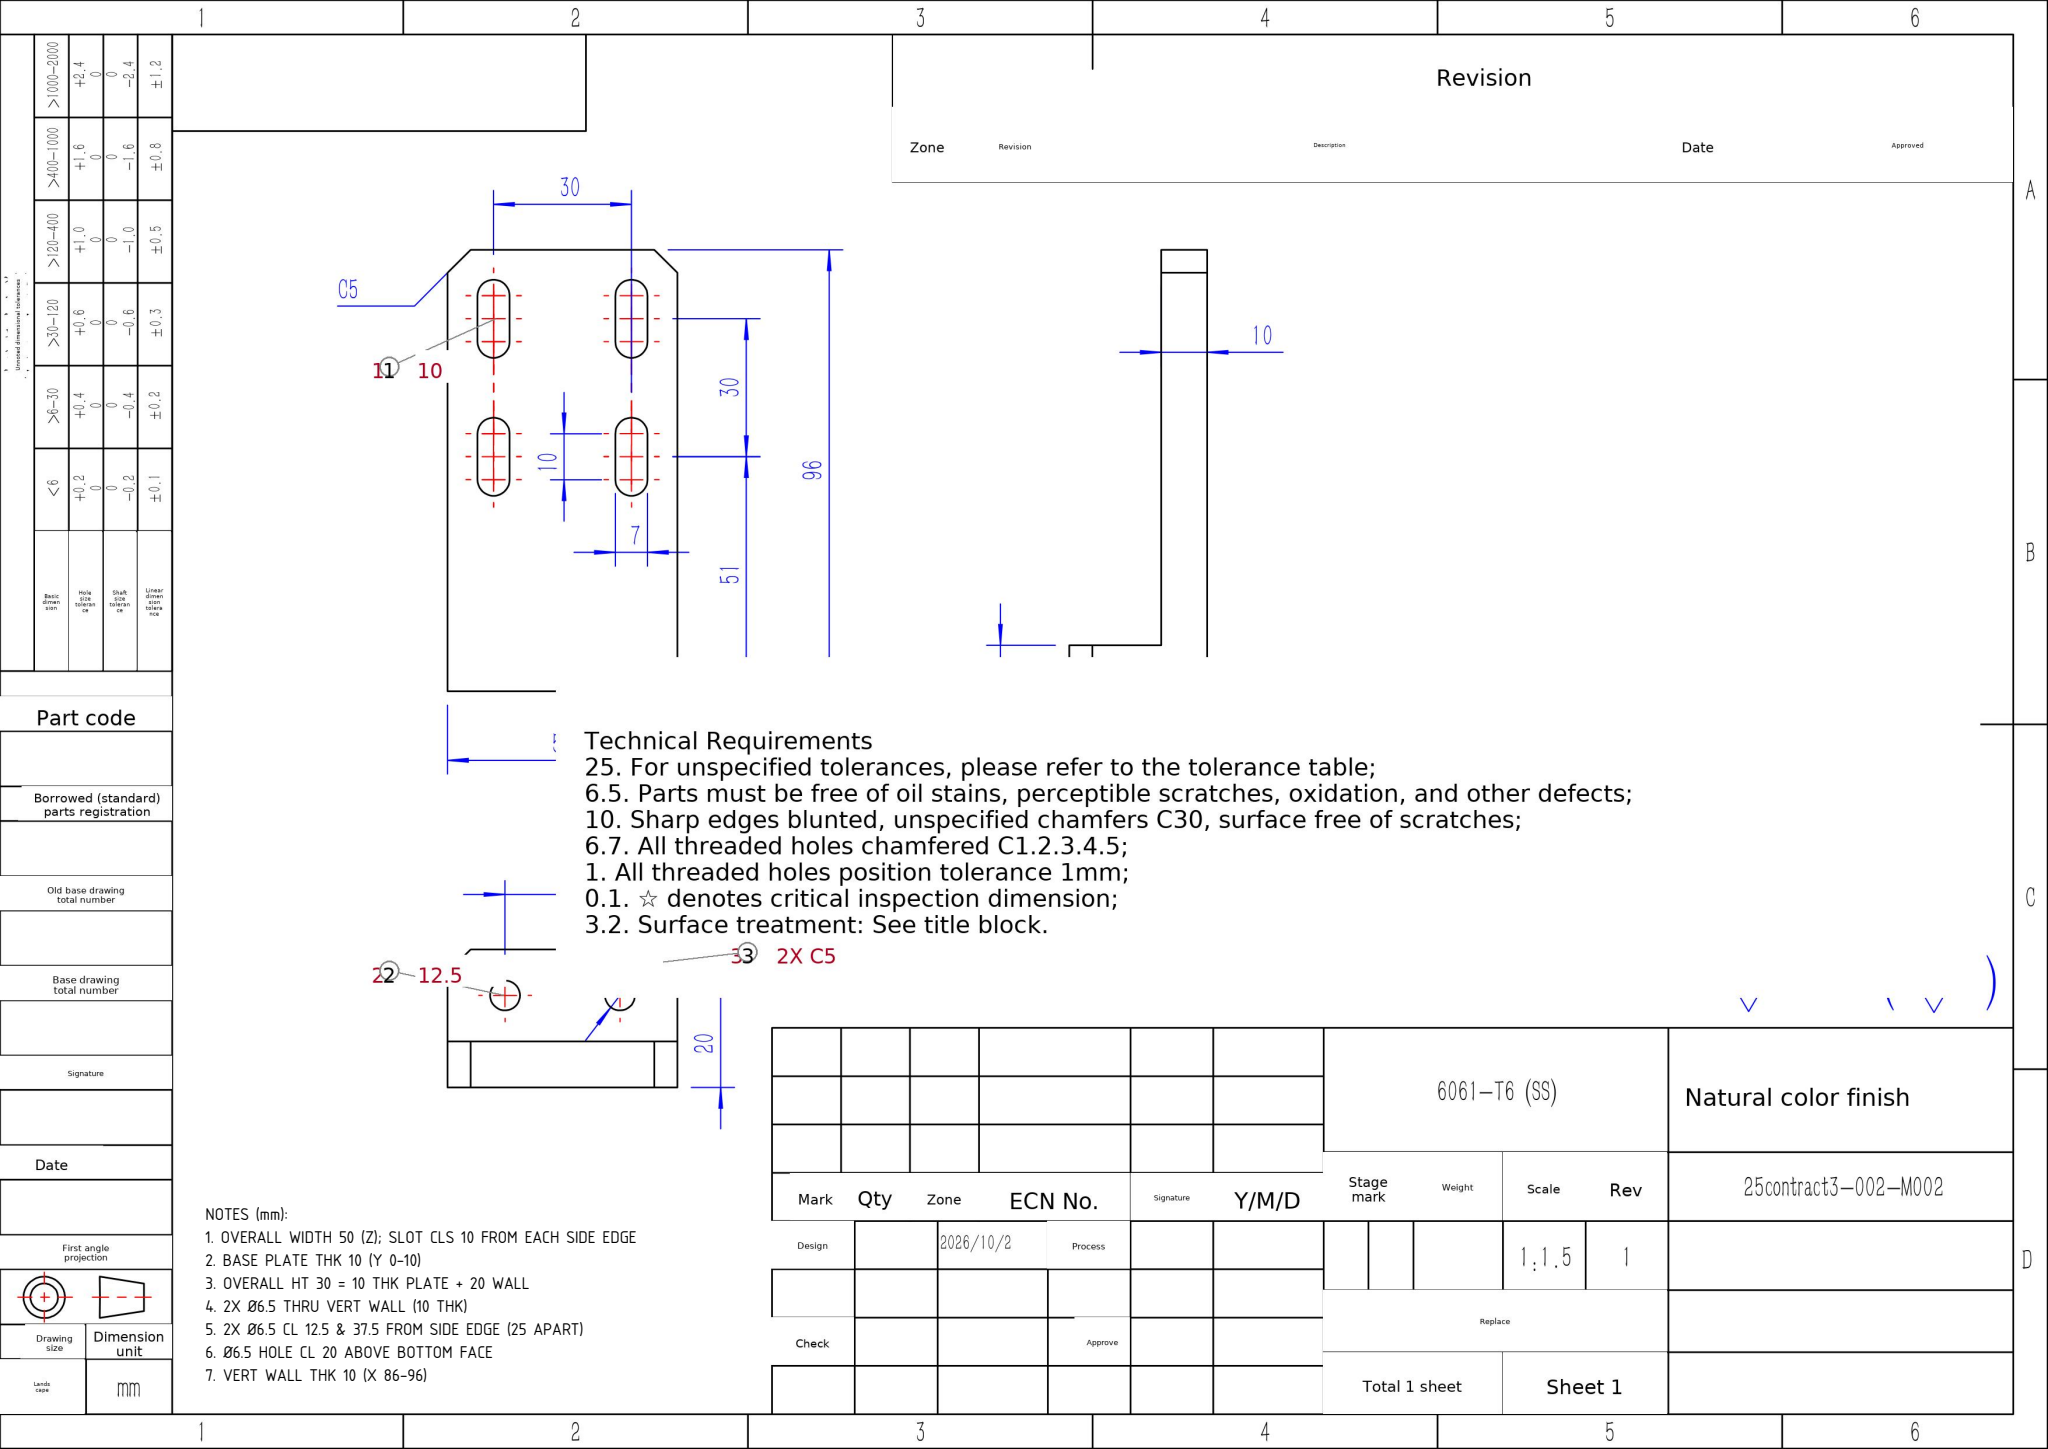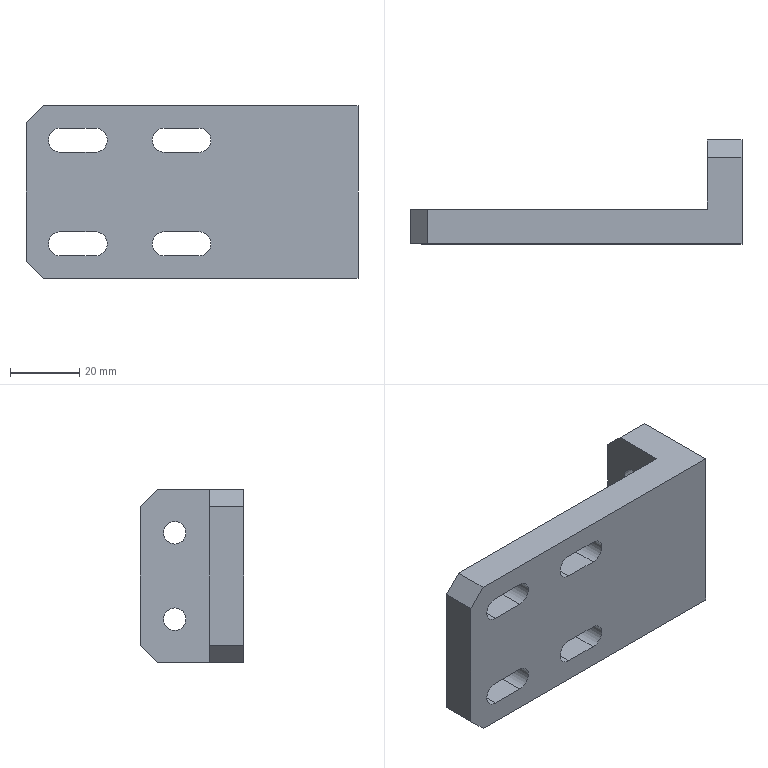Part | SolidWorks | mm | 1 solid | 32 faces | box 96 x 30 x 50 mm | volume 52497 mm3 | plane 20 | cylinder 12 | commonest cylinder face diameters 7 x8 6.5 x4
Drawing notes:
OVERALL WIDTH 50 (Z); SLOT CLS 10 FROM EACH SIDE EDGE | from the solid: bbox Z=50; Ø7 slot axes at z=10 and z=40
BASE PLATE THK 10 (Y 0-10) | from the solid: y planes at 0 and 10; Ø7 slots length 10
OVERALL HT 30 = 10 THK PLATE + 20 WALL | from the solid: y planes 0, 10, 30; bbox Y=30
2X Ø6.5 THRU VERT WALL (10 THK) | from the solid: cyl dia 6.5, axis x, length 10, x wall 86-96
2X Ø6.5 CL 12.5 & 37.5 FROM SIDE EDGE (25 APART) | from the solid: cyl dia 6.5 at z=12.5 and z=37.5
Ø6.5 HOLE CL 20 ABOVE BOTTOM FACE | from the solid: cyl dia 6.5 at y=20; bottom face y=0
VERT WALL THK 10 (X 86-96) | from the solid: x planes at 86.0 and 96.0
STEP:
#1=CARTESIAN_POINT('',(48.,20.,9.25));
#2=VERTEX_POINT('',#1);
#3=CARTESIAN_POINT('',(48.,20.,15.75));
#4=VERTEX_POINT('',#3);
#5=CARTESIAN_POINT('',(48.,20.,12.5));
#6=DIRECTION('',(-1.,0.,-0.));
#7=DIRECTION('',(0.,0.,1.));
#8=AXIS2_PLACEMENT_3D('',#5,#6,#7);
#9=CIRCLE('',#8,3.25);
#10=EDGE_CURVE('',#2,#4,#9,.T.);
#11=ORIENTED_EDGE('',*,*,#10,.F.);
#12=CARTESIAN_POINT('',(38.,20.,9.25));
#13=VERTEX_POINT('',#12);
#14=CARTESIAN_POINT('',(38.,20.,9.25));
#15=DIRECTION('',(-1.,0.,-0.));
#16=VECTOR('',#15,1000.);
#17=LINE('',#14,#16);
#18=EDGE_CURVE('',#2,#13,#17,.T.);
#19=ORIENTED_EDGE('',*,*,#18,.T.);
#20=CARTESIAN_POINT('',(38.,20.,15.75));
#21=VERTEX_POINT('',#20);
#22=CARTESIAN_POINT('',(38.,20.,12.5));
#23=DIRECTION('',(-1.,0.,-0.));
#24=DIRECTION('',(0.,0.,1.));
#25=AXIS2_PLACEMENT_3D('',#22,#23,#24);
#26=CIRCLE('',#25,3.25);
#27=EDGE_CURVE('',#13,#21,#26,.T.);
#28=ORIENTED_EDGE('',*,*,#27,.T.);
#29=CARTESIAN_POINT('',(38.,20.,15.75));
#30=DIRECTION('',(-1.,0.,-0.));
#31=VECTOR('',#30,1000.);
#32=LINE('',#29,#31);
#33=EDGE_CURVE('',#4,#21,#32,.T.);
#34=ORIENTED_EDGE('',*,*,#33,.F.);
#35=EDGE_LOOP('',(#11,#19,#28,#34));
#36=FACE_OUTER_BOUND('',#35,.T.);
#37=CARTESIAN_POINT('',(38.,20.,12.5));
#38=DIRECTION('',(-1.,0.,-0.));
#39=DIRECTION('',(0.,0.,1.));
#40=AXIS2_PLACEMENT_3D('',#37,#38,#39);
#41=CYLINDRICAL_SURFACE('',#40,3.25);
#42=ADVANCED_FACE('',(#36),#41,.F.);
#43=CARTESIAN_POINT('',(48.,20.,-15.75));
#44=VERTEX_POINT('',#43);
#45=CARTESIAN_POINT('',(48.,20.,-9.25));
#46=VERTEX_POINT('',#45);
#47=CARTESIAN_POINT('',(48.,20.,-12.5));
#48=DIRECTION('',(-1.,0.,-0.));
#49=DIRECTION('',(0.,0.,1.));
#50=AXIS2_PLACEMENT_3D('',#47,#48,#49);
#51=CIRCLE('',#50,3.25);
#52=EDGE_CURVE('',#44,#46,#51,.T.);
#53=ORIENTED_EDGE('',*,*,#52,.F.);
#54=CARTESIAN_POINT('',(38.,20.,-15.75));
#55=VERTEX_POINT('',#54);
#56=CARTESIAN_POINT('',(38.,20.,-15.75));
#57=DIRECTION('',(-1.,0.,-0.));
#58=VECTOR('',#57,1000.);
#59=LINE('',#56,#58);
#60=EDGE_CURVE('',#44,#55,#59,.T.);
#61=ORIENTED_EDGE('',*,*,#60,.T.);
#62=CARTESIAN_POINT('',(38.,20.,-9.25));
#63=VERTEX_POINT('',#62);
#64=CARTESIAN_POINT('',(38.,20.,-12.5));
#65=DIRECTION('',(-1.,0.,-0.));
#66=DIRECTION('',(0.,0.,1.));
#67=AXIS2_PLACEMENT_3D('',#64,#65,#66);
#68=CIRCLE('',#67,3.25);
#69=EDGE_CURVE('',#55,#63,#68,.T.);
#70=ORIENTED_EDGE('',*,*,#69,.T.);
#71=CARTESIAN_POINT('',(38.,20.,-9.25));
#72=DIRECTION('',(-1.,0.,-0.));
#73=VECTOR('',#72,1000.);
#74=LINE('',#71,#73);
#75=EDGE_CURVE('',#46,#63,#74,.T.);
#76=ORIENTED_EDGE('',*,*,#75,.F.);
#77=EDGE_LOOP('',(#53,#61,#70,#76));
#78=FACE_OUTER_BOUND('',#77,.T.);
#79=CARTESIAN_POINT('',(38.,20.,-12.5));
#80=DIRECTION('',(-1.,0.,-0.));
#81=DIRECTION('',(0.,0.,1.));
#82=AXIS2_PLACEMENT_3D('',#79,#80,#81);
#83=CYLINDRICAL_SURFACE('',#82,3.25);
#84=ADVANCED_FACE('',(#78),#83,.F.);
#85=CARTESIAN_POINT('',(48.,20.,12.5));
#86=DIRECTION('',(-1.,0.,-0.));
#87=DIRECTION('',(0.,0.,1.));
#88=AXIS2_PLACEMENT_3D('',#85,#86,#87);
#89=CIRCLE('',#88,3.25);
#90=EDGE_CURVE('',#4,#2,#89,.T.);
#91=ORIENTED_EDGE('',*,*,#90,.T.);
#92=ORIENTED_EDGE('',*,*,#10,.T.);
#93=EDGE_LOOP('',(#91,#92));
#94=FACE_BOUND('',#93,.T.);
#95=CARTESIAN_POINT('',(48.,20.,-12.5));
#96=DIRECTION('',(-1.,0.,-0.));
#97=DIRECTION('',(0.,0.,1.));
#98=AXIS2_PLACEMENT_3D('',#95,#96,#97);
#99=CIRCLE('',#98,3.25);
#100=EDGE_CURVE('',#46,#44,#99,.T.);
#101=ORIENTED_EDGE('',*,*,#100,.T.);
#102=ORIENTED_EDGE('',*,*,#52,.T.);
#103=EDGE_LOOP('',(#101,#102));
#104=FACE_BOUND('',#103,.T.);
#105=CARTESIAN_POINT('',(48.,30.,-20.));
#106=VERTEX_POINT('',#105);
#107=CARTESIAN_POINT('',(48.,30.,20.));
#108=VERTEX_POINT('',#107);
#109=CARTESIAN_POINT('',(48.,30.,-25.));
#110=DIRECTION('',(0.,0.,1.));
#111=VECTOR('',#110,1000.);
#112=LINE('',#109,#111);
#113=EDGE_CURVE('',#106,#108,#112,.T.);
#114=ORIENTED_EDGE('',*,*,#113,.T.);
#115=CARTESIAN_POINT('',(48.,25.,25.));
#116=VERTEX_POINT('',#115);
#117=CARTESIAN_POINT('',(48.,25.,25.));
#118=DIRECTION('',(0.,-0.7071,0.7071));
#119=VECTOR('',#118,1000.);
#120=LINE('',#117,#119);
#121=EDGE_CURVE('',#108,#116,#120,.T.);
#122=ORIENTED_EDGE('',*,*,#121,.T.);
#123=CARTESIAN_POINT('',(48.,0.,25.));
#124=VERTEX_POINT('',#123);
#125=CARTESIAN_POINT('',(48.,10.,25.));
#126=DIRECTION('',(0.,-1.,0.));
#127=VECTOR('',#126,1000.);
#128=LINE('',#125,#127);
#129=EDGE_CURVE('',#116,#124,#128,.T.);
#130=ORIENTED_EDGE('',*,*,#129,.T.);
#131=CARTESIAN_POINT('',(48.,0.,-25.));
#132=VERTEX_POINT('',#131);
#133=CARTESIAN_POINT('',(48.,0.,25.));
#134=DIRECTION('',(0.,0.,-1.));
#135=VECTOR('',#134,1000.);
#136=LINE('',#133,#135);
#137=EDGE_CURVE('',#124,#132,#136,.T.);
#138=ORIENTED_EDGE('',*,*,#137,.T.);
#139=CARTESIAN_POINT('',(48.,25.,-25.));
#140=VERTEX_POINT('',#139);
#141=CARTESIAN_POINT('',(48.,10.,-25.));
#142=DIRECTION('',(0.,-1.,0.));
#143=VECTOR('',#142,1000.);
#144=LINE('',#141,#143);
#145=EDGE_CURVE('',#140,#132,#144,.T.);
#146=ORIENTED_EDGE('',*,*,#145,.F.);
#147=CARTESIAN_POINT('',(48.,25.,-25.));
#148=DIRECTION('',(0.,0.7071,0.7071));
#149=VECTOR('',#148,1000.);
#150=LINE('',#147,#149);
#151=EDGE_CURVE('',#140,#106,#150,.T.);
#152=ORIENTED_EDGE('',*,*,#151,.T.);
#153=EDGE_LOOP('',(#114,#122,#130,#138,#146,#152));
#154=FACE_OUTER_BOUND('',#153,.T.);
#155=CARTESIAN_POINT('',(48.,10.,25.));
#156=DIRECTION('',(-1.,0.,0.));
#157=DIRECTION('',(0.,0.,1.));
#158=AXIS2_PLACEMENT_3D('',#155,#156,#157);
#159=PLANE('',#158);
#160=ADVANCED_FACE('',(#94,#104,#154),#159,.F.);
#161=CARTESIAN_POINT('',(38.,25.,-25.));
#162=VERTEX_POINT('',#161);
#163=CARTESIAN_POINT('',(38.,10.,-25.));
#164=VERTEX_POINT('',#163);
#165=CARTESIAN_POINT('',(38.,30.,-25.));
#166=DIRECTION('',(0.,-1.,0.));
#167=VECTOR('',#166,1000.);
#168=LINE('',#165,#167);
#169=EDGE_CURVE('',#162,#164,#168,.T.);
#170=ORIENTED_EDGE('',*,*,#169,.F.);
#171=CARTESIAN_POINT('',(-48.,25.,-25.));
#172=DIRECTION('',(1.,0.,0.));
#173=VECTOR('',#172,1000.);
#174=LINE('',#171,#173);
#175=EDGE_CURVE('',#162,#140,#174,.T.);
#176=ORIENTED_EDGE('',*,*,#175,.T.);
#177=ORIENTED_EDGE('',*,*,#145,.T.);
#178=CARTESIAN_POINT('',(-43.,0.,-25.));
#179=VERTEX_POINT('',#178);
#180=CARTESIAN_POINT('',(-48.,0.,-25.));
#181=DIRECTION('',(-1.,0.,0.));
#182=VECTOR('',#181,1000.);
#183=LINE('',#180,#182);
#184=EDGE_CURVE('',#132,#179,#183,.T.);
#185=ORIENTED_EDGE('',*,*,#184,.T.);
#186=CARTESIAN_POINT('',(-43.,10.,-25.));
#187=VERTEX_POINT('',#186);
#188=CARTESIAN_POINT('',(-43.,10.,-25.));
#189=DIRECTION('',(0.,1.,0.));
#190=VECTOR('',#189,1000.);
#191=LINE('',#188,#190);
#192=EDGE_CURVE('',#179,#187,#191,.T.);
#193=ORIENTED_EDGE('',*,*,#192,.T.);
#194=CARTESIAN_POINT('',(-48.,10.,-25.));
#195=DIRECTION('',(-1.,0.,0.));
#196=VECTOR('',#195,1000.);
#197=LINE('',#194,#196);
#198=EDGE_CURVE('',#164,#187,#197,.T.);
#199=ORIENTED_EDGE('',*,*,#198,.F.);
#200=EDGE_LOOP('',(#170,#176,#177,#185,#193,#199));
#201=FACE_OUTER_BOUND('',#200,.T.);
#202=CARTESIAN_POINT('',(-48.,10.,-25.));
#203=DIRECTION('',(0.,0.,1.));
#204=DIRECTION('',(1.,0.,0.));
#205=AXIS2_PLACEMENT_3D('',#202,#203,#204);
#206=PLANE('',#205);
#207=ADVANCED_FACE('',(#201),#206,.F.);
#208=CARTESIAN_POINT('',(-48.,10.,-20.));
#209=VERTEX_POINT('',#208);
#210=CARTESIAN_POINT('',(-48.,10.,20.));
#211=VERTEX_POINT('',#210);
#212=CARTESIAN_POINT('',(-48.,10.,25.));
#213=DIRECTION('',(0.,0.,1.));
#214=VECTOR('',#213,1000.);
#215=LINE('',#212,#214);
#216=EDGE_CURVE('',#209,#211,#215,.T.);
#217=ORIENTED_EDGE('',*,*,#216,.F.);
#218=CARTESIAN_POINT('',(-48.,0.,-20.));
#219=VERTEX_POINT('',#218);
#220=CARTESIAN_POINT('',(-48.,10.,-20.));
#221=DIRECTION('',(0.,-1.,0.));
#222=VECTOR('',#221,1000.);
#223=LINE('',#220,#222);
#224=EDGE_CURVE('',#209,#219,#223,.T.);
#225=ORIENTED_EDGE('',*,*,#224,.T.);
#226=CARTESIAN_POINT('',(-48.,0.,20.));
#227=VERTEX_POINT('',#226);
#228=CARTESIAN_POINT('',(-48.,0.,25.));
#229=DIRECTION('',(0.,0.,1.));
#230=VECTOR('',#229,1000.);
#231=LINE('',#228,#230);
#232=EDGE_CURVE('',#219,#227,#231,.T.);
#233=ORIENTED_EDGE('',*,*,#232,.T.);
#234=CARTESIAN_POINT('',(-48.,10.,20.));
#235=DIRECTION('',(0.,1.,0.));
#236=VECTOR('',#235,1000.);
#237=LINE('',#234,#236);
#238=EDGE_CURVE('',#227,#211,#237,.T.);
#239=ORIENTED_EDGE('',*,*,#238,.T.);
#240=EDGE_LOOP('',(#217,#225,#233,#239));
#241=FACE_OUTER_BOUND('',#240,.T.);
#242=CARTESIAN_POINT('',(-48.,10.,25.));
#243=DIRECTION('',(1.,0.,0.));
#244=DIRECTION('',(0.,0.,-1.));
#245=AXIS2_PLACEMENT_3D('',#242,#243,#244);
#246=PLANE('',#245);
#247=ADVANCED_FACE('',(#241),#246,.F.);
#248=ORIENTED_EDGE('',*,*,#129,.F.);
#249=CARTESIAN_POINT('',(38.,25.,25.));
#250=VERTEX_POINT('',#249);
#251=CARTESIAN_POINT('',(-48.,25.,25.));
#252=DIRECTION('',(-1.,0.,0.));
#253=VECTOR('',#252,1000.);
#254=LINE('',#251,#253);
#255=EDGE_CURVE('',#116,#250,#254,.T.);
#256=ORIENTED_EDGE('',*,*,#255,.T.);
#257=CARTESIAN_POINT('',(38.,10.,25.));
#258=VERTEX_POINT('',#257);
#259=CARTESIAN_POINT('',(38.,30.,25.));
#260=DIRECTION('',(0.,-1.,0.));
#261=VECTOR('',#260,1000.);
#262=LINE('',#259,#261);
#263=EDGE_CURVE('',#250,#258,#262,.T.);
#264=ORIENTED_EDGE('',*,*,#263,.T.);
#265=CARTESIAN_POINT('',(-43.,10.,25.));
#266=VERTEX_POINT('',#265);
#267=CARTESIAN_POINT('',(-48.,10.,25.));
#268=DIRECTION('',(1.,0.,0.));
#269=VECTOR('',#268,1000.);
#270=LINE('',#267,#269);
#271=EDGE_CURVE('',#266,#258,#270,.T.);
#272=ORIENTED_EDGE('',*,*,#271,.F.);
#273=CARTESIAN_POINT('',(-43.,0.,25.));
#274=VERTEX_POINT('',#273);
#275=CARTESIAN_POINT('',(-43.,10.,25.));
#276=DIRECTION('',(0.,-1.,0.));
#277=VECTOR('',#276,1000.);
#278=LINE('',#275,#277);
#279=EDGE_CURVE('',#266,#274,#278,.T.);
#280=ORIENTED_EDGE('',*,*,#279,.T.);
#281=CARTESIAN_POINT('',(-48.,0.,25.));
#282=DIRECTION('',(1.,0.,0.));
#283=VECTOR('',#282,1000.);
#284=LINE('',#281,#283);
#285=EDGE_CURVE('',#274,#124,#284,.T.);
#286=ORIENTED_EDGE('',*,*,#285,.T.);
#287=EDGE_LOOP('',(#248,#256,#264,#272,#280,#286));
#288=FACE_OUTER_BOUND('',#287,.T.);
#289=CARTESIAN_POINT('',(-48.,10.,25.));
#290=DIRECTION('',(0.,0.,-1.));
#291=DIRECTION('',(-1.,0.,0.));
#292=AXIS2_PLACEMENT_3D('',#289,#290,#291);
#293=PLANE('',#292);
#294=ADVANCED_FACE('',(#288),#293,.F.);
#295=CARTESIAN_POINT('',(-8.,10.,18.5));
#296=VERTEX_POINT('',#295);
#297=CARTESIAN_POINT('',(2.,10.,18.5));
#298=VERTEX_POINT('',#297);
#299=CARTESIAN_POINT('',(-8.,10.,18.5));
#300=DIRECTION('',(1.,0.,0.));
#301=VECTOR('',#300,1000.);
#302=LINE('',#299,#301);
#303=EDGE_CURVE('',#296,#298,#302,.T.);
#304=ORIENTED_EDGE('',*,*,#303,.F.);
#305=CARTESIAN_POINT('',(-8.,10.,11.5));
#306=VERTEX_POINT('',#305);
#307=CARTESIAN_POINT('',(-8.,10.,15.));
#308=DIRECTION('',(0.,1.,0.));
#309=DIRECTION('',(0.,0.,1.));
#310=AXIS2_PLACEMENT_3D('',#307,#308,#309);
#311=CIRCLE('',#310,3.5);
#312=EDGE_CURVE('',#306,#296,#311,.T.);
#313=ORIENTED_EDGE('',*,*,#312,.F.);
#314=CARTESIAN_POINT('',(2.,10.,11.5));
#315=VERTEX_POINT('',#314);
#316=CARTESIAN_POINT('',(-8.,10.,11.5));
#317=DIRECTION('',(-1.,0.,0.));
#318=VECTOR('',#317,1000.);
#319=LINE('',#316,#318);
#320=EDGE_CURVE('',#315,#306,#319,.T.);
#321=ORIENTED_EDGE('',*,*,#320,.F.);
#322=CARTESIAN_POINT('',(2.,10.,15.));
#323=DIRECTION('',(0.,1.,0.));
#324=DIRECTION('',(0.,0.,1.));
#325=AXIS2_PLACEMENT_3D('',#322,#323,#324);
#326=CIRCLE('',#325,3.5);
#327=EDGE_CURVE('',#298,#315,#326,.T.);
#328=ORIENTED_EDGE('',*,*,#327,.F.);
#329=EDGE_LOOP('',(#304,#313,#321,#328));
#330=FACE_BOUND('',#329,.T.);
#331=CARTESIAN_POINT('',(-8.,10.,-11.5));
#332=VERTEX_POINT('',#331);
#333=CARTESIAN_POINT('',(2.,10.,-11.5));
#334=VERTEX_POINT('',#333);
#335=CARTESIAN_POINT('',(-8.,10.,-11.5));
#336=DIRECTION('',(1.,0.,0.));
#337=VECTOR('',#336,1000.);
#338=LINE('',#335,#337);
#339=EDGE_CURVE('',#332,#334,#338,.T.);
#340=ORIENTED_EDGE('',*,*,#339,.F.);
#341=CARTESIAN_POINT('',(-8.,10.,-18.5));
#342=VERTEX_POINT('',#341);
#343=CARTESIAN_POINT('',(-8.,10.,-15.));
#344=DIRECTION('',(0.,1.,0.));
#345=DIRECTION('',(0.,0.,-1.));
#346=AXIS2_PLACEMENT_3D('',#343,#344,#345);
#347=CIRCLE('',#346,3.5);
#348=EDGE_CURVE('',#342,#332,#347,.T.);
#349=ORIENTED_EDGE('',*,*,#348,.F.);
#350=CARTESIAN_POINT('',(2.,10.,-18.5));
#351=VERTEX_POINT('',#350);
#352=CARTESIAN_POINT('',(-8.,10.,-18.5));
#353=DIRECTION('',(-1.,0.,0.));
#354=VECTOR('',#353,1000.);
#355=LINE('',#352,#354);
#356=EDGE_CURVE('',#351,#342,#355,.T.);
#357=ORIENTED_EDGE('',*,*,#356,.F.);
#358=CARTESIAN_POINT('',(2.,10.,-15.));
#359=DIRECTION('',(0.,1.,0.));
#360=DIRECTION('',(0.,0.,-1.));
#361=AXIS2_PLACEMENT_3D('',#358,#359,#360);
#362=CIRCLE('',#361,3.5);
#363=EDGE_CURVE('',#334,#351,#362,.T.);
#364=ORIENTED_EDGE('',*,*,#363,.F.);
#365=EDGE_LOOP('',(#340,#349,#357,#364));
#366=FACE_BOUND('',#365,.T.);
#367=CARTESIAN_POINT('',(-38.,10.,18.5));
#368=VERTEX_POINT('',#367);
#369=CARTESIAN_POINT('',(-28.,10.,18.5));
#370=VERTEX_POINT('',#369);
#371=CARTESIAN_POINT('',(-38.,10.,18.5));
#372=DIRECTION('',(1.,0.,0.));
#373=VECTOR('',#372,1000.);
#374=LINE('',#371,#373);
#375=EDGE_CURVE('',#368,#370,#374,.T.);
#376=ORIENTED_EDGE('',*,*,#375,.F.);
#377=CARTESIAN_POINT('',(-38.,10.,11.5));
#378=VERTEX_POINT('',#377);
#379=CARTESIAN_POINT('',(-38.,10.,15.));
#380=DIRECTION('',(0.,1.,0.));
#381=DIRECTION('',(0.,0.,1.));
#382=AXIS2_PLACEMENT_3D('',#379,#380,#381);
#383=CIRCLE('',#382,3.5);
#384=EDGE_CURVE('',#378,#368,#383,.T.);
#385=ORIENTED_EDGE('',*,*,#384,.F.);
#386=CARTESIAN_POINT('',(-28.,10.,11.5));
#387=VERTEX_POINT('',#386);
#388=CARTESIAN_POINT('',(-38.,10.,11.5));
#389=DIRECTION('',(-1.,0.,0.));
#390=VECTOR('',#389,1000.);
#391=LINE('',#388,#390);
#392=EDGE_CURVE('',#387,#378,#391,.T.);
#393=ORIENTED_EDGE('',*,*,#392,.F.);
#394=CARTESIAN_POINT('',(-28.,10.,15.));
#395=DIRECTION('',(0.,1.,0.));
#396=DIRECTION('',(0.,0.,1.));
#397=AXIS2_PLACEMENT_3D('',#394,#395,#396);
#398=CIRCLE('',#397,3.5);
#399=EDGE_CURVE('',#370,#387,#398,.T.);
#400=ORIENTED_EDGE('',*,*,#399,.F.);
#401=EDGE_LOOP('',(#376,#385,#393,#400));
#402=FACE_BOUND('',#401,.T.);
#403=CARTESIAN_POINT('',(-38.,10.,-11.5));
#404=VERTEX_POINT('',#403);
#405=CARTESIAN_POINT('',(-28.,10.,-11.5));
#406=VERTEX_POINT('',#405);
#407=CARTESIAN_POINT('',(-38.,10.,-11.5));
#408=DIRECTION('',(1.,0.,0.));
#409=VECTOR('',#408,1000.);
#410=LINE('',#407,#409);
#411=EDGE_CURVE('',#404,#406,#410,.T.);
#412=ORIENTED_EDGE('',*,*,#411,.F.);
#413=CARTESIAN_POINT('',(-38.,10.,-18.5));
#414=VERTEX_POINT('',#413);
#415=CARTESIAN_POINT('',(-38.,10.,-15.));
#416=DIRECTION('',(0.,1.,0.));
#417=DIRECTION('',(0.,0.,-1.));
#418=AXIS2_PLACEMENT_3D('',#415,#416,#417);
#419=CIRCLE('',#418,3.5);
#420=EDGE_CURVE('',#414,#404,#419,.T.);
#421=ORIENTED_EDGE('',*,*,#420,.F.);
#422=CARTESIAN_POINT('',(-28.,10.,-18.5));
#423=VERTEX_POINT('',#422);
#424=CARTESIAN_POINT('',(-38.,10.,-18.5));
#425=DIRECTION('',(-1.,0.,0.));
#426=VECTOR('',#425,1000.);
#427=LINE('',#424,#426);
#428=EDGE_CURVE('',#423,#414,#427,.T.);
#429=ORIENTED_EDGE('',*,*,#428,.F.);
#430=CARTESIAN_POINT('',(-28.,10.,-15.));
#431=DIRECTION('',(0.,1.,0.));
#432=DIRECTION('',(0.,0.,-1.));
#433=AXIS2_PLACEMENT_3D('',#430,#431,#432);
#434=CIRCLE('',#433,3.5);
#435=EDGE_CURVE('',#406,#423,#434,.T.);
#436=ORIENTED_EDGE('',*,*,#435,.F.);
#437=EDGE_LOOP('',(#412,#421,#429,#436));
#438=FACE_BOUND('',#437,.T.);
#439=ORIENTED_EDGE('',*,*,#198,.T.);
#440=CARTESIAN_POINT('',(-48.,10.,-20.));
#441=DIRECTION('',(-0.7071,0.,0.7071));
#442=VECTOR('',#441,1000.);
#443=LINE('',#440,#442);
#444=EDGE_CURVE('',#187,#209,#443,.T.);
#445=ORIENTED_EDGE('',*,*,#444,.T.);
#446=ORIENTED_EDGE('',*,*,#216,.T.);
#447=CARTESIAN_POINT('',(-43.,10.,25.));
#448=DIRECTION('',(0.7071,0.,0.7071));
#449=VECTOR('',#448,1000.);
#450=LINE('',#447,#449);
#451=EDGE_CURVE('',#211,#266,#450,.T.);
#452=ORIENTED_EDGE('',*,*,#451,.T.);
#453=ORIENTED_EDGE('',*,*,#271,.T.);
#454=CARTESIAN_POINT('',(38.,10.,0.));
#455=DIRECTION('',(0.,0.,-1.));
#456=VECTOR('',#455,1000.);
#457=LINE('',#454,#456);
#458=EDGE_CURVE('',#258,#164,#457,.T.);
#459=ORIENTED_EDGE('',*,*,#458,.T.);
#460=EDGE_LOOP('',(#439,#445,#446,#452,#453,#459));
#461=FACE_OUTER_BOUND('',#460,.T.);
#462=CARTESIAN_POINT('',(0.,10.,0.));
#463=DIRECTION('',(0.,-1.,0.));
#464=DIRECTION('',(0.,0.,-1.));
#465=AXIS2_PLACEMENT_3D('',#462,#463,#464);
#466=PLANE('',#465);
#467=ADVANCED_FACE('',(#330,#366,#402,#438,#461),#466,.F.);
#468=CARTESIAN_POINT('',(-8.,0.,11.5));
#469=VERTEX_POINT('',#468);
#470=CARTESIAN_POINT('',(-8.,0.,18.5));
#471=VERTEX_POINT('',#470);
#472=CARTESIAN_POINT('',(-8.,0.,15.));
#473=DIRECTION('',(0.,1.,0.));
#474=DIRECTION('',(0.,0.,1.));
#475=AXIS2_PLACEMENT_3D('',#472,#473,#474);
#476=CIRCLE('',#475,3.5);
#477=EDGE_CURVE('',#469,#471,#476,.T.);
#478=ORIENTED_EDGE('',*,*,#477,.T.);
#479=CARTESIAN_POINT('',(2.,0.,18.5));
#480=VERTEX_POINT('',#479);
#481=CARTESIAN_POINT('',(-8.,0.,18.5));
#482=DIRECTION('',(1.,0.,0.));
#483=VECTOR('',#482,1000.);
#484=LINE('',#481,#483);
#485=EDGE_CURVE('',#471,#480,#484,.T.);
#486=ORIENTED_EDGE('',*,*,#485,.T.);
#487=CARTESIAN_POINT('',(2.,0.,11.5));
#488=VERTEX_POINT('',#487);
#489=CARTESIAN_POINT('',(2.,0.,15.));
#490=DIRECTION('',(0.,1.,0.));
#491=DIRECTION('',(0.,0.,1.));
#492=AXIS2_PLACEMENT_3D('',#489,#490,#491);
#493=CIRCLE('',#492,3.5);
#494=EDGE_CURVE('',#480,#488,#493,.T.);
#495=ORIENTED_EDGE('',*,*,#494,.T.);
#496=CARTESIAN_POINT('',(-8.,0.,11.5));
#497=DIRECTION('',(-1.,0.,0.));
#498=VECTOR('',#497,1000.);
#499=LINE('',#496,#498);
#500=EDGE_CURVE('',#488,#469,#499,.T.);
#501=ORIENTED_EDGE('',*,*,#500,.T.);
#502=EDGE_LOOP('',(#478,#486,#495,#501));
#503=FACE_BOUND('',#502,.T.);
#504=CARTESIAN_POINT('',(-8.,0.,-18.5));
#505=VERTEX_POINT('',#504);
#506=CARTESIAN_POINT('',(-8.,0.,-11.5));
#507=VERTEX_POINT('',#506);
#508=CARTESIAN_POINT('',(-8.,0.,-15.));
#509=DIRECTION('',(0.,1.,0.));
#510=DIRECTION('',(0.,0.,-1.));
#511=AXIS2_PLACEMENT_3D('',#508,#509,#510);
#512=CIRCLE('',#511,3.5);
#513=EDGE_CURVE('',#505,#507,#512,.T.);
#514=ORIENTED_EDGE('',*,*,#513,.T.);
#515=CARTESIAN_POINT('',(2.,0.,-11.5));
#516=VERTEX_POINT('',#515);
#517=CARTESIAN_POINT('',(-8.,0.,-11.5));
#518=DIRECTION('',(1.,0.,0.));
#519=VECTOR('',#518,1000.);
#520=LINE('',#517,#519);
#521=EDGE_CURVE('',#507,#516,#520,.T.);
#522=ORIENTED_EDGE('',*,*,#521,.T.);
#523=CARTESIAN_POINT('',(2.,0.,-18.5));
#524=VERTEX_POINT('',#523);
#525=CARTESIAN_POINT('',(2.,0.,-15.));
#526=DIRECTION('',(0.,1.,0.));
#527=DIRECTION('',(0.,0.,-1.));
#528=AXIS2_PLACEMENT_3D('',#525,#526,#527);
#529=CIRCLE('',#528,3.5);
#530=EDGE_CURVE('',#516,#524,#529,.T.);
#531=ORIENTED_EDGE('',*,*,#530,.T.);
#532=CARTESIAN_POINT('',(-8.,0.,-18.5));
#533=DIRECTION('',(-1.,0.,0.));
#534=VECTOR('',#533,1000.);
#535=LINE('',#532,#534);
#536=EDGE_CURVE('',#524,#505,#535,.T.);
#537=ORIENTED_EDGE('',*,*,#536,.T.);
#538=EDGE_LOOP('',(#514,#522,#531,#537));
#539=FACE_BOUND('',#538,.T.);
#540=CARTESIAN_POINT('',(-38.,0.,11.5));
#541=VERTEX_POINT('',#540);
#542=CARTESIAN_POINT('',(-38.,0.,18.5));
#543=VERTEX_POINT('',#542);
#544=CARTESIAN_POINT('',(-38.,0.,15.));
#545=DIRECTION('',(0.,1.,0.));
#546=DIRECTION('',(0.,0.,1.));
#547=AXIS2_PLACEMENT_3D('',#544,#545,#546);
#548=CIRCLE('',#547,3.5);
#549=EDGE_CURVE('',#541,#543,#548,.T.);
#550=ORIENTED_EDGE('',*,*,#549,.T.);
#551=CARTESIAN_POINT('',(-28.,0.,18.5));
#552=VERTEX_POINT('',#551);
#553=CARTESIAN_POINT('',(-38.,0.,18.5));
#554=DIRECTION('',(1.,0.,0.));
#555=VECTOR('',#554,1000.);
#556=LINE('',#553,#555);
#557=EDGE_CURVE('',#543,#552,#556,.T.);
#558=ORIENTED_EDGE('',*,*,#557,.T.);
#559=CARTESIAN_POINT('',(-28.,0.,11.5));
#560=VERTEX_POINT('',#559);
#561=CARTESIAN_POINT('',(-28.,0.,15.));
#562=DIRECTION('',(0.,1.,0.));
#563=DIRECTION('',(0.,0.,1.));
#564=AXIS2_PLACEMENT_3D('',#561,#562,#563);
#565=CIRCLE('',#564,3.5);
#566=EDGE_CURVE('',#552,#560,#565,.T.);
#567=ORIENTED_EDGE('',*,*,#566,.T.);
#568=CARTESIAN_POINT('',(-38.,0.,11.5));
#569=DIRECTION('',(-1.,0.,0.));
#570=VECTOR('',#569,1000.);
#571=LINE('',#568,#570);
#572=EDGE_CURVE('',#560,#541,#571,.T.);
#573=ORIENTED_EDGE('',*,*,#572,.T.);
#574=EDGE_LOOP('',(#550,#558,#567,#573));
#575=FACE_BOUND('',#574,.T.);
#576=CARTESIAN_POINT('',(-38.,0.,-18.5));
#577=VERTEX_POINT('',#576);
#578=CARTESIAN_POINT('',(-38.,0.,-11.5));
#579=VERTEX_POINT('',#578);
#580=CARTESIAN_POINT('',(-38.,0.,-15.));
#581=DIRECTION('',(0.,1.,0.));
#582=DIRECTION('',(0.,0.,-1.));
#583=AXIS2_PLACEMENT_3D('',#580,#581,#582);
#584=CIRCLE('',#583,3.5);
#585=EDGE_CURVE('',#577,#579,#584,.T.);
#586=ORIENTED_EDGE('',*,*,#585,.T.);
#587=CARTESIAN_POINT('',(-28.,0.,-11.5));
#588=VERTEX_POINT('',#587);
#589=CARTESIAN_POINT('',(-38.,0.,-11.5));
#590=DIRECTION('',(1.,0.,0.));
#591=VECTOR('',#590,1000.);
#592=LINE('',#589,#591);
#593=EDGE_CURVE('',#579,#588,#592,.T.);
#594=ORIENTED_EDGE('',*,*,#593,.T.);
#595=CARTESIAN_POINT('',(-28.,0.,-18.5));
#596=VERTEX_POINT('',#595);
#597=CARTESIAN_POINT('',(-28.,0.,-15.));
#598=DIRECTION('',(0.,1.,0.));
#599=DIRECTION('',(0.,0.,-1.));
#600=AXIS2_PLACEMENT_3D('',#597,#598,#599);
#601=CIRCLE('',#600,3.5);
#602=EDGE_CURVE('',#588,#596,#601,.T.);
#603=ORIENTED_EDGE('',*,*,#602,.T.);
#604=CARTESIAN_POINT('',(-38.,0.,-18.5));
#605=DIRECTION('',(-1.,0.,0.));
#606=VECTOR('',#605,1000.);
#607=LINE('',#604,#606);
#608=EDGE_CURVE('',#596,#577,#607,.T.);
#609=ORIENTED_EDGE('',*,*,#608,.T.);
#610=EDGE_LOOP('',(#586,#594,#603,#609));
#611=FACE_BOUND('',#610,.T.);
#612=ORIENTED_EDGE('',*,*,#232,.F.);
#613=CARTESIAN_POINT('',(-34.,0.,-34.));
#614=DIRECTION('',(0.7071,0.,-0.7071));
#615=VECTOR('',#614,1000.);
#616=LINE('',#613,#615);
#617=EDGE_CURVE('',#219,#179,#616,.T.);
#618=ORIENTED_EDGE('',*,*,#617,.T.);
#619=ORIENTED_EDGE('',*,*,#184,.F.);
#620=ORIENTED_EDGE('',*,*,#137,.F.);
#621=ORIENTED_EDGE('',*,*,#285,.F.);
#622=CARTESIAN_POINT('',(-34.,0.,34.));
#623=DIRECTION('',(-0.7071,0.,-0.7071));
#624=VECTOR('',#623,1000.);
#625=LINE('',#622,#624);
#626=EDGE_CURVE('',#274,#227,#625,.T.);
#627=ORIENTED_EDGE('',*,*,#626,.T.);
#628=EDGE_LOOP('',(#612,#618,#619,#620,#621,#627));
#629=FACE_OUTER_BOUND('',#628,.T.);
#630=CARTESIAN_POINT('',(0.,0.,0.));
#631=DIRECTION('',(0.,-1.,0.));
#632=DIRECTION('',(0.,0.,-1.));
#633=AXIS2_PLACEMENT_3D('',#630,#631,#632);
#634=PLANE('',#633);
#635=ADVANCED_FACE('',(#503,#539,#575,#611,#629),#634,.T.);
#636=CARTESIAN_POINT('',(38.,20.,12.5));
#637=DIRECTION('',(-1.,0.,-0.));
#638=DIRECTION('',(0.,0.,1.));
#639=AXIS2_PLACEMENT_3D('',#636,#637,#638);
#640=CIRCLE('',#639,3.25);
#641=EDGE_CURVE('',#21,#13,#640,.T.);
#642=ORIENTED_EDGE('',*,*,#641,.F.);
#643=ORIENTED_EDGE('',*,*,#27,.F.);
#644=EDGE_LOOP('',(#642,#643));
#645=FACE_BOUND('',#644,.T.);
#646=CARTESIAN_POINT('',(38.,20.,-12.5));
#647=DIRECTION('',(-1.,0.,-0.));
#648=DIRECTION('',(0.,0.,1.));
#649=AXIS2_PLACEMENT_3D('',#646,#647,#648);
#650=CIRCLE('',#649,3.25);
#651=EDGE_CURVE('',#63,#55,#650,.T.);
#652=ORIENTED_EDGE('',*,*,#651,.F.);
#653=ORIENTED_EDGE('',*,*,#69,.F.);
#654=EDGE_LOOP('',(#652,#653));
#655=FACE_BOUND('',#654,.T.);
#656=ORIENTED_EDGE('',*,*,#263,.F.);
#657=CARTESIAN_POINT('',(38.,30.,20.));
#658=VERTEX_POINT('',#657);
#659=CARTESIAN_POINT('',(38.,52.5,-2.5));
#660=DIRECTION('',(0.,0.7071,-0.7071));
#661=VECTOR('',#660,1000.);
#662=LINE('',#659,#661);
#663=EDGE_CURVE('',#250,#658,#662,.T.);
#664=ORIENTED_EDGE('',*,*,#663,.T.);
#665=CARTESIAN_POINT('',(38.,30.,-20.));
#666=VERTEX_POINT('',#665);
#667=CARTESIAN_POINT('',(38.,30.,-25.));
#668=DIRECTION('',(0.,0.,-1.));
#669=VECTOR('',#668,1000.);
#670=LINE('',#667,#669);
#671=EDGE_CURVE('',#658,#666,#670,.T.);
#672=ORIENTED_EDGE('',*,*,#671,.T.);
#673=CARTESIAN_POINT('',(38.,27.5,-22.5));
#674=DIRECTION('',(0.,-0.7071,-0.7071));
#675=VECTOR('',#674,1000.);
#676=LINE('',#673,#675);
#677=EDGE_CURVE('',#666,#162,#676,.T.);
#678=ORIENTED_EDGE('',*,*,#677,.T.);
#679=ORIENTED_EDGE('',*,*,#169,.T.);
#680=ORIENTED_EDGE('',*,*,#458,.F.);
#681=EDGE_LOOP('',(#656,#664,#672,#678,#679,#680));
#682=FACE_OUTER_BOUND('',#681,.T.);
#683=CARTESIAN_POINT('',(38.,30.,-25.));
#684=DIRECTION('',(-1.,0.,-0.));
#685=DIRECTION('',(-0.,0.,1.));
#686=AXIS2_PLACEMENT_3D('',#683,#684,#685);
#687=PLANE('',#686);
#688=ADVANCED_FACE('',(#645,#655,#682),#687,.T.);
#689=ORIENTED_EDGE('',*,*,#671,.F.);
#690=CARTESIAN_POINT('',(0.,30.,20.));
#691=DIRECTION('',(1.,0.,0.));
#692=VECTOR('',#691,1000.);
#693=LINE('',#690,#692);
#694=EDGE_CURVE('',#658,#108,#693,.T.);
#695=ORIENTED_EDGE('',*,*,#694,.T.);
#696=ORIENTED_EDGE('',*,*,#113,.F.);
#697=CARTESIAN_POINT('',(0.,30.,-20.));
#698=DIRECTION('',(-1.,0.,0.));
#699=VECTOR('',#698,1000.);
#700=LINE('',#697,#699);
#701=EDGE_CURVE('',#106,#666,#700,.T.);
#702=ORIENTED_EDGE('',*,*,#701,.T.);
#703=EDGE_LOOP('',(#689,#695,#696,#702));
#704=FACE_OUTER_BOUND('',#703,.T.);
#705=CARTESIAN_POINT('',(0.,30.,0.));
#706=DIRECTION('',(0.,-1.,0.));
#707=DIRECTION('',(0.,0.,-1.));
#708=AXIS2_PLACEMENT_3D('',#705,#706,#707);
#709=PLANE('',#708);
#710=ADVANCED_FACE('',(#704),#709,.F.);
#711=ORIENTED_EDGE('',*,*,#121,.F.);
#712=ORIENTED_EDGE('',*,*,#694,.F.);
#713=ORIENTED_EDGE('',*,*,#663,.F.);
#714=ORIENTED_EDGE('',*,*,#255,.F.);
#715=EDGE_LOOP('',(#711,#712,#713,#714));
#716=FACE_OUTER_BOUND('',#715,.T.);
#717=CARTESIAN_POINT('',(-48.,25.,25.));
#718=DIRECTION('',(0.,-0.7071,-0.7071));
#719=DIRECTION('',(-1.,0.,0.));
#720=AXIS2_PLACEMENT_3D('',#717,#718,#719);
#721=PLANE('',#720);
#722=ADVANCED_FACE('',(#716),#721,.F.);
#723=ORIENTED_EDGE('',*,*,#677,.F.);
#724=ORIENTED_EDGE('',*,*,#701,.F.);
#725=ORIENTED_EDGE('',*,*,#151,.F.);
#726=ORIENTED_EDGE('',*,*,#175,.F.);
#727=EDGE_LOOP('',(#723,#724,#725,#726));
#728=FACE_OUTER_BOUND('',#727,.T.);
#729=CARTESIAN_POINT('',(-48.,25.,-25.));
#730=DIRECTION('',(0.,-0.7071,0.7071));
#731=DIRECTION('',(1.,0.,0.));
#732=AXIS2_PLACEMENT_3D('',#729,#730,#731);
#733=PLANE('',#732);
#734=ADVANCED_FACE('',(#728),#733,.F.);
#735=ORIENTED_EDGE('',*,*,#444,.F.);
#736=ORIENTED_EDGE('',*,*,#192,.F.);
#737=ORIENTED_EDGE('',*,*,#617,.F.);
#738=ORIENTED_EDGE('',*,*,#224,.F.);
#739=EDGE_LOOP('',(#735,#736,#737,#738));
#740=FACE_OUTER_BOUND('',#739,.T.);
#741=CARTESIAN_POINT('',(-48.,10.,-20.));
#742=DIRECTION('',(0.7071,0.,0.7071));
#743=DIRECTION('',(0.,-1.,0.));
#744=AXIS2_PLACEMENT_3D('',#741,#742,#743);
#745=PLANE('',#744);
#746=ADVANCED_FACE('',(#740),#745,.F.);
#747=ORIENTED_EDGE('',*,*,#451,.F.);
#748=ORIENTED_EDGE('',*,*,#238,.F.);
#749=ORIENTED_EDGE('',*,*,#626,.F.);
#750=ORIENTED_EDGE('',*,*,#279,.F.);
#751=EDGE_LOOP('',(#747,#748,#749,#750));
#752=FACE_OUTER_BOUND('',#751,.T.);
#753=CARTESIAN_POINT('',(-43.,10.,25.));
#754=DIRECTION('',(0.7071,0.,-0.7071));
#755=DIRECTION('',(0.,-1.,0.));
#756=AXIS2_PLACEMENT_3D('',#753,#754,#755);
#757=PLANE('',#756);
#758=ADVANCED_FACE('',(#752),#757,.F.);
#759=ORIENTED_EDGE('',*,*,#60,.F.);
#760=ORIENTED_EDGE('',*,*,#100,.F.);
#761=ORIENTED_EDGE('',*,*,#75,.T.);
#762=ORIENTED_EDGE('',*,*,#651,.T.);
#763=EDGE_LOOP('',(#759,#760,#761,#762));
#764=FACE_OUTER_BOUND('',#763,.T.);
#765=CARTESIAN_POINT('',(38.,20.,-12.5));
#766=DIRECTION('',(-1.,0.,-0.));
#767=DIRECTION('',(0.,0.,1.));
#768=AXIS2_PLACEMENT_3D('',#765,#766,#767);
#769=CYLINDRICAL_SURFACE('',#768,3.25);
#770=ADVANCED_FACE('',(#764),#769,.F.);
#771=ORIENTED_EDGE('',*,*,#18,.F.);
#772=ORIENTED_EDGE('',*,*,#90,.F.);
#773=ORIENTED_EDGE('',*,*,#33,.T.);
#774=ORIENTED_EDGE('',*,*,#641,.T.);
#775=EDGE_LOOP('',(#771,#772,#773,#774));
#776=FACE_OUTER_BOUND('',#775,.T.);
#777=CARTESIAN_POINT('',(38.,20.,12.5));
#778=DIRECTION('',(-1.,0.,-0.));
#779=DIRECTION('',(0.,0.,1.));
#780=AXIS2_PLACEMENT_3D('',#777,#778,#779);
#781=CYLINDRICAL_SURFACE('',#780,3.25);
#782=ADVANCED_FACE('',(#776),#781,.F.);
#783=ORIENTED_EDGE('',*,*,#420,.T.);
#784=CARTESIAN_POINT('',(-38.,0.,-11.5));
#785=DIRECTION('',(0.,1.,0.));
#786=VECTOR('',#785,1000.);
#787=LINE('',#784,#786);
#788=EDGE_CURVE('',#579,#404,#787,.T.);
#789=ORIENTED_EDGE('',*,*,#788,.F.);
#790=ORIENTED_EDGE('',*,*,#585,.F.);
#791=CARTESIAN_POINT('',(-38.,0.,-18.5));
#792=DIRECTION('',(0.,1.,0.));
#793=VECTOR('',#792,1000.);
#794=LINE('',#791,#793);
#795=EDGE_CURVE('',#577,#414,#794,.T.);
#796=ORIENTED_EDGE('',*,*,#795,.T.);
#797=EDGE_LOOP('',(#783,#789,#790,#796));
#798=FACE_OUTER_BOUND('',#797,.T.);
#799=CARTESIAN_POINT('',(-38.,0.,-15.));
#800=DIRECTION('',(0.,1.,0.));
#801=DIRECTION('',(0.,0.,1.));
#802=AXIS2_PLACEMENT_3D('',#799,#800,#801);
#803=CYLINDRICAL_SURFACE('',#802,3.5);
#804=ADVANCED_FACE('',(#798),#803,.F.);
#805=ORIENTED_EDGE('',*,*,#428,.T.);
#806=ORIENTED_EDGE('',*,*,#795,.F.);
#807=ORIENTED_EDGE('',*,*,#608,.F.);
#808=CARTESIAN_POINT('',(-28.,0.,-18.5));
#809=DIRECTION('',(0.,1.,0.));
#810=VECTOR('',#809,1000.);
#811=LINE('',#808,#810);
#812=EDGE_CURVE('',#596,#423,#811,.T.);
#813=ORIENTED_EDGE('',*,*,#812,.T.);
#814=EDGE_LOOP('',(#805,#806,#807,#813));
#815=FACE_OUTER_BOUND('',#814,.T.);
#816=CARTESIAN_POINT('',(-38.,0.,-18.5));
#817=DIRECTION('',(0.,0.,-1.));
#818=DIRECTION('',(-1.,0.,0.));
#819=AXIS2_PLACEMENT_3D('',#816,#817,#818);
#820=PLANE('',#819);
#821=ADVANCED_FACE('',(#815),#820,.F.);
#822=ORIENTED_EDGE('',*,*,#435,.T.);
#823=ORIENTED_EDGE('',*,*,#812,.F.);
#824=ORIENTED_EDGE('',*,*,#602,.F.);
#825=CARTESIAN_POINT('',(-28.,0.,-11.5));
#826=DIRECTION('',(0.,1.,0.));
#827=VECTOR('',#826,1000.);
#828=LINE('',#825,#827);
#829=EDGE_CURVE('',#588,#406,#828,.T.);
#830=ORIENTED_EDGE('',*,*,#829,.T.);
#831=EDGE_LOOP('',(#822,#823,#824,#830));
#832=FACE_OUTER_BOUND('',#831,.T.);
#833=CARTESIAN_POINT('',(-28.,0.,-15.));
#834=DIRECTION('',(0.,1.,0.));
#835=DIRECTION('',(0.,0.,1.));
#836=AXIS2_PLACEMENT_3D('',#833,#834,#835);
#837=CYLINDRICAL_SURFACE('',#836,3.5);
#838=ADVANCED_FACE('',(#832),#837,.F.);
#839=ORIENTED_EDGE('',*,*,#411,.T.);
#840=ORIENTED_EDGE('',*,*,#829,.F.);
#841=ORIENTED_EDGE('',*,*,#593,.F.);
#842=ORIENTED_EDGE('',*,*,#788,.T.);
#843=EDGE_LOOP('',(#839,#840,#841,#842));
#844=FACE_OUTER_BOUND('',#843,.T.);
#845=CARTESIAN_POINT('',(-38.,0.,-11.5));
#846=DIRECTION('',(0.,0.,1.));
#847=DIRECTION('',(1.,0.,0.));
#848=AXIS2_PLACEMENT_3D('',#845,#846,#847);
#849=PLANE('',#848);
#850=ADVANCED_FACE('',(#844),#849,.F.);
#851=ORIENTED_EDGE('',*,*,#384,.T.);
#852=CARTESIAN_POINT('',(-38.,0.,18.5));
#853=DIRECTION('',(0.,1.,0.));
#854=VECTOR('',#853,1000.);
#855=LINE('',#852,#854);
#856=EDGE_CURVE('',#543,#368,#855,.T.);
#857=ORIENTED_EDGE('',*,*,#856,.F.);
#858=ORIENTED_EDGE('',*,*,#549,.F.);
#859=CARTESIAN_POINT('',(-38.,0.,11.5));
#860=DIRECTION('',(0.,1.,0.));
#861=VECTOR('',#860,1000.);
#862=LINE('',#859,#861);
#863=EDGE_CURVE('',#541,#378,#862,.T.);
#864=ORIENTED_EDGE('',*,*,#863,.T.);
#865=EDGE_LOOP('',(#851,#857,#858,#864));
#866=FACE_OUTER_BOUND('',#865,.T.);
#867=CARTESIAN_POINT('',(-38.,0.,15.));
#868=DIRECTION('',(0.,1.,0.));
#869=DIRECTION('',(0.,0.,1.));
#870=AXIS2_PLACEMENT_3D('',#867,#868,#869);
#871=CYLINDRICAL_SURFACE('',#870,3.5);
#872=ADVANCED_FACE('',(#866),#871,.F.);
#873=ORIENTED_EDGE('',*,*,#392,.T.);
#874=ORIENTED_EDGE('',*,*,#863,.F.);
#875=ORIENTED_EDGE('',*,*,#572,.F.);
#876=CARTESIAN_POINT('',(-28.,0.,11.5));
#877=DIRECTION('',(0.,1.,0.));
#878=VECTOR('',#877,1000.);
#879=LINE('',#876,#878);
#880=EDGE_CURVE('',#560,#387,#879,.T.);
#881=ORIENTED_EDGE('',*,*,#880,.T.);
#882=EDGE_LOOP('',(#873,#874,#875,#881));
#883=FACE_OUTER_BOUND('',#882,.T.);
#884=CARTESIAN_POINT('',(-38.,0.,11.5));
#885=DIRECTION('',(0.,0.,-1.));
#886=DIRECTION('',(-1.,0.,0.));
#887=AXIS2_PLACEMENT_3D('',#884,#885,#886);
#888=PLANE('',#887);
#889=ADVANCED_FACE('',(#883),#888,.F.);
#890=ORIENTED_EDGE('',*,*,#399,.T.);
#891=ORIENTED_EDGE('',*,*,#880,.F.);
#892=ORIENTED_EDGE('',*,*,#566,.F.);
#893=CARTESIAN_POINT('',(-28.,0.,18.5));
#894=DIRECTION('',(0.,1.,0.));
#895=VECTOR('',#894,1000.);
#896=LINE('',#893,#895);
#897=EDGE_CURVE('',#552,#370,#896,.T.);
#898=ORIENTED_EDGE('',*,*,#897,.T.);
#899=EDGE_LOOP('',(#890,#891,#892,#898));
#900=FACE_OUTER_BOUND('',#899,.T.);
#901=CARTESIAN_POINT('',(-28.,0.,15.));
#902=DIRECTION('',(0.,1.,0.));
#903=DIRECTION('',(0.,0.,1.));
#904=AXIS2_PLACEMENT_3D('',#901,#902,#903);
#905=CYLINDRICAL_SURFACE('',#904,3.5);
#906=ADVANCED_FACE('',(#900),#905,.F.);
#907=ORIENTED_EDGE('',*,*,#375,.T.);
#908=ORIENTED_EDGE('',*,*,#897,.F.);
#909=ORIENTED_EDGE('',*,*,#557,.F.);
#910=ORIENTED_EDGE('',*,*,#856,.T.);
#911=EDGE_LOOP('',(#907,#908,#909,#910));
#912=FACE_OUTER_BOUND('',#911,.T.);
#913=CARTESIAN_POINT('',(-38.,0.,18.5));
#914=DIRECTION('',(0.,0.,1.));
#915=DIRECTION('',(1.,0.,0.));
#916=AXIS2_PLACEMENT_3D('',#913,#914,#915);
#917=PLANE('',#916);
#918=ADVANCED_FACE('',(#912),#917,.F.);
#919=ORIENTED_EDGE('',*,*,#348,.T.);
#920=CARTESIAN_POINT('',(-8.,0.,-11.5));
#921=DIRECTION('',(0.,1.,0.));
#922=VECTOR('',#921,1000.);
#923=LINE('',#920,#922);
#924=EDGE_CURVE('',#507,#332,#923,.T.);
#925=ORIENTED_EDGE('',*,*,#924,.F.);
#926=ORIENTED_EDGE('',*,*,#513,.F.);
#927=CARTESIAN_POINT('',(-8.,0.,-18.5));
#928=DIRECTION('',(0.,1.,0.));
#929=VECTOR('',#928,1000.);
#930=LINE('',#927,#929);
#931=EDGE_CURVE('',#505,#342,#930,.T.);
#932=ORIENTED_EDGE('',*,*,#931,.T.);
#933=EDGE_LOOP('',(#919,#925,#926,#932));
#934=FACE_OUTER_BOUND('',#933,.T.);
#935=CARTESIAN_POINT('',(-8.,0.,-15.));
#936=DIRECTION('',(0.,1.,0.));
#937=DIRECTION('',(0.,0.,1.));
#938=AXIS2_PLACEMENT_3D('',#935,#936,#937);
#939=CYLINDRICAL_SURFACE('',#938,3.5);
#940=ADVANCED_FACE('',(#934),#939,.F.);
#941=ORIENTED_EDGE('',*,*,#356,.T.);
#942=ORIENTED_EDGE('',*,*,#931,.F.);
#943=ORIENTED_EDGE('',*,*,#536,.F.);
#944=CARTESIAN_POINT('',(2.,0.,-18.5));
#945=DIRECTION('',(0.,1.,0.));
#946=VECTOR('',#945,1000.);
#947=LINE('',#944,#946);
#948=EDGE_CURVE('',#524,#351,#947,.T.);
#949=ORIENTED_EDGE('',*,*,#948,.T.);
#950=EDGE_LOOP('',(#941,#942,#943,#949));
#951=FACE_OUTER_BOUND('',#950,.T.);
#952=CARTESIAN_POINT('',(-8.,0.,-18.5));
#953=DIRECTION('',(0.,0.,-1.));
#954=DIRECTION('',(-1.,0.,0.));
#955=AXIS2_PLACEMENT_3D('',#952,#953,#954);
#956=PLANE('',#955);
#957=ADVANCED_FACE('',(#951),#956,.F.);
#958=ORIENTED_EDGE('',*,*,#363,.T.);
#959=ORIENTED_EDGE('',*,*,#948,.F.);
#960=ORIENTED_EDGE('',*,*,#530,.F.);
#961=CARTESIAN_POINT('',(2.,0.,-11.5));
#962=DIRECTION('',(0.,1.,0.));
#963=VECTOR('',#962,1000.);
#964=LINE('',#961,#963);
#965=EDGE_CURVE('',#516,#334,#964,.T.);
#966=ORIENTED_EDGE('',*,*,#965,.T.);
#967=EDGE_LOOP('',(#958,#959,#960,#966));
#968=FACE_OUTER_BOUND('',#967,.T.);
#969=CARTESIAN_POINT('',(2.,0.,-15.));
#970=DIRECTION('',(0.,1.,0.));
#971=DIRECTION('',(0.,0.,1.));
#972=AXIS2_PLACEMENT_3D('',#969,#970,#971);
#973=CYLINDRICAL_SURFACE('',#972,3.5);
#974=ADVANCED_FACE('',(#968),#973,.F.);
#975=ORIENTED_EDGE('',*,*,#339,.T.);
#976=ORIENTED_EDGE('',*,*,#965,.F.);
#977=ORIENTED_EDGE('',*,*,#521,.F.);
#978=ORIENTED_EDGE('',*,*,#924,.T.);
#979=EDGE_LOOP('',(#975,#976,#977,#978));
#980=FACE_OUTER_BOUND('',#979,.T.);
#981=CARTESIAN_POINT('',(-8.,0.,-11.5));
#982=DIRECTION('',(0.,0.,1.));
#983=DIRECTION('',(1.,0.,0.));
#984=AXIS2_PLACEMENT_3D('',#981,#982,#983);
#985=PLANE('',#984);
#986=ADVANCED_FACE('',(#980),#985,.F.);
#987=ORIENTED_EDGE('',*,*,#312,.T.);
#988=CARTESIAN_POINT('',(-8.,0.,18.5));
#989=DIRECTION('',(0.,1.,0.));
#990=VECTOR('',#989,1000.);
#991=LINE('',#988,#990);
#992=EDGE_CURVE('',#471,#296,#991,.T.);
#993=ORIENTED_EDGE('',*,*,#992,.F.);
#994=ORIENTED_EDGE('',*,*,#477,.F.);
#995=CARTESIAN_POINT('',(-8.,0.,11.5));
#996=DIRECTION('',(0.,1.,0.));
#997=VECTOR('',#996,1000.);
#998=LINE('',#995,#997);
#999=EDGE_CURVE('',#469,#306,#998,.T.);
#1000=ORIENTED_EDGE('',*,*,#999,.T.);
#1001=EDGE_LOOP('',(#987,#993,#994,#1000));
#1002=FACE_OUTER_BOUND('',#1001,.T.);
#1003=CARTESIAN_POINT('',(-8.,0.,15.));
#1004=DIRECTION('',(0.,1.,0.));
#1005=DIRECTION('',(0.,0.,1.));
#1006=AXIS2_PLACEMENT_3D('',#1003,#1004,#1005);
#1007=CYLINDRICAL_SURFACE('',#1006,3.5);
#1008=ADVANCED_FACE('',(#1002),#1007,.F.);
#1009=ORIENTED_EDGE('',*,*,#320,.T.);
#1010=ORIENTED_EDGE('',*,*,#999,.F.);
#1011=ORIENTED_EDGE('',*,*,#500,.F.);
#1012=CARTESIAN_POINT('',(2.,0.,11.5));
#1013=DIRECTION('',(0.,1.,0.));
#1014=VECTOR('',#1013,1000.);
#1015=LINE('',#1012,#1014);
#1016=EDGE_CURVE('',#488,#315,#1015,.T.);
#1017=ORIENTED_EDGE('',*,*,#1016,.T.);
#1018=EDGE_LOOP('',(#1009,#1010,#1011,#1017));
#1019=FACE_OUTER_BOUND('',#1018,.T.);
#1020=CARTESIAN_POINT('',(-8.,0.,11.5));
#1021=DIRECTION('',(0.,0.,-1.));
#1022=DIRECTION('',(-1.,0.,0.));
#1023=AXIS2_PLACEMENT_3D('',#1020,#1021,#1022);
#1024=PLANE('',#1023);
#1025=ADVANCED_FACE('',(#1019),#1024,.F.);
#1026=ORIENTED_EDGE('',*,*,#327,.T.);
#1027=ORIENTED_EDGE('',*,*,#1016,.F.);
#1028=ORIENTED_EDGE('',*,*,#494,.F.);
#1029=CARTESIAN_POINT('',(2.,0.,18.5));
#1030=DIRECTION('',(0.,1.,0.));
#1031=VECTOR('',#1030,1000.);
#1032=LINE('',#1029,#1031);
#1033=EDGE_CURVE('',#480,#298,#1032,.T.);
#1034=ORIENTED_EDGE('',*,*,#1033,.T.);
#1035=EDGE_LOOP('',(#1026,#1027,#1028,#1034));
#1036=FACE_OUTER_BOUND('',#1035,.T.);
#1037=CARTESIAN_POINT('',(2.,0.,15.));
#1038=DIRECTION('',(0.,1.,0.));
#1039=DIRECTION('',(0.,0.,1.));
#1040=AXIS2_PLACEMENT_3D('',#1037,#1038,#1039);
#1041=CYLINDRICAL_SURFACE('',#1040,3.5);
#1042=ADVANCED_FACE('',(#1036),#1041,.F.);
#1043=ORIENTED_EDGE('',*,*,#303,.T.);
#1044=ORIENTED_EDGE('',*,*,#1033,.F.);
#1045=ORIENTED_EDGE('',*,*,#485,.F.);
#1046=ORIENTED_EDGE('',*,*,#992,.T.);
#1047=EDGE_LOOP('',(#1043,#1044,#1045,#1046));
#1048=FACE_OUTER_BOUND('',#1047,.T.);
#1049=CARTESIAN_POINT('',(-8.,0.,18.5));
#1050=DIRECTION('',(0.,0.,1.));
#1051=DIRECTION('',(1.,0.,0.));
#1052=AXIS2_PLACEMENT_3D('',#1049,#1050,#1051);
#1053=PLANE('',#1052);
#1054=ADVANCED_FACE('',(#1048),#1053,.F.);
#1055=CLOSED_SHELL('',(#42,#84,#160,#207,#247,#294,#467,#635,#688,#710,#722,#734,#746,#758,#770,#782,#804,#821,#838,#850,#872,#889,#906,#918,#940,#957,#974,#986,#1008,#1025,#1042,#1054));
#1056=MANIFOLD_SOLID_BREP('',#1055);
#1057=CARTESIAN_POINT('',(0.,0.,0.));
#1058=DIRECTION('',(0.,0.,1.));
#1059=DIRECTION('',(1.,0.,0.));
#1060=AXIS2_PLACEMENT_3D('',#1057,#1058,#1059);
#1061=(LENGTH_UNIT()NAMED_UNIT(*)SI_UNIT(.MILLI.,.METRE.));
#1062=UNCERTAINTY_MEASURE_WITH_UNIT(LENGTH_MEASURE(0.00001),#1061,'','');
#1063=(NAMED_UNIT(*)PLANE_ANGLE_UNIT()SI_UNIT($,.RADIAN.));
#1064=(NAMED_UNIT(*)SI_UNIT($,.STERADIAN.)SOLID_ANGLE_UNIT());
#1065=(GEOMETRIC_REPRESENTATION_CONTEXT(3)GLOBAL_UNCERTAINTY_ASSIGNED_CONTEXT((#1062))GLOBAL_UNIT_ASSIGNED_CONTEXT((#1061,#1063,#1064))REPRESENTATION_CONTEXT('',''));
#1066=ADVANCED_BREP_SHAPE_REPRESENTATION('',(#1056,#1060),#1065);